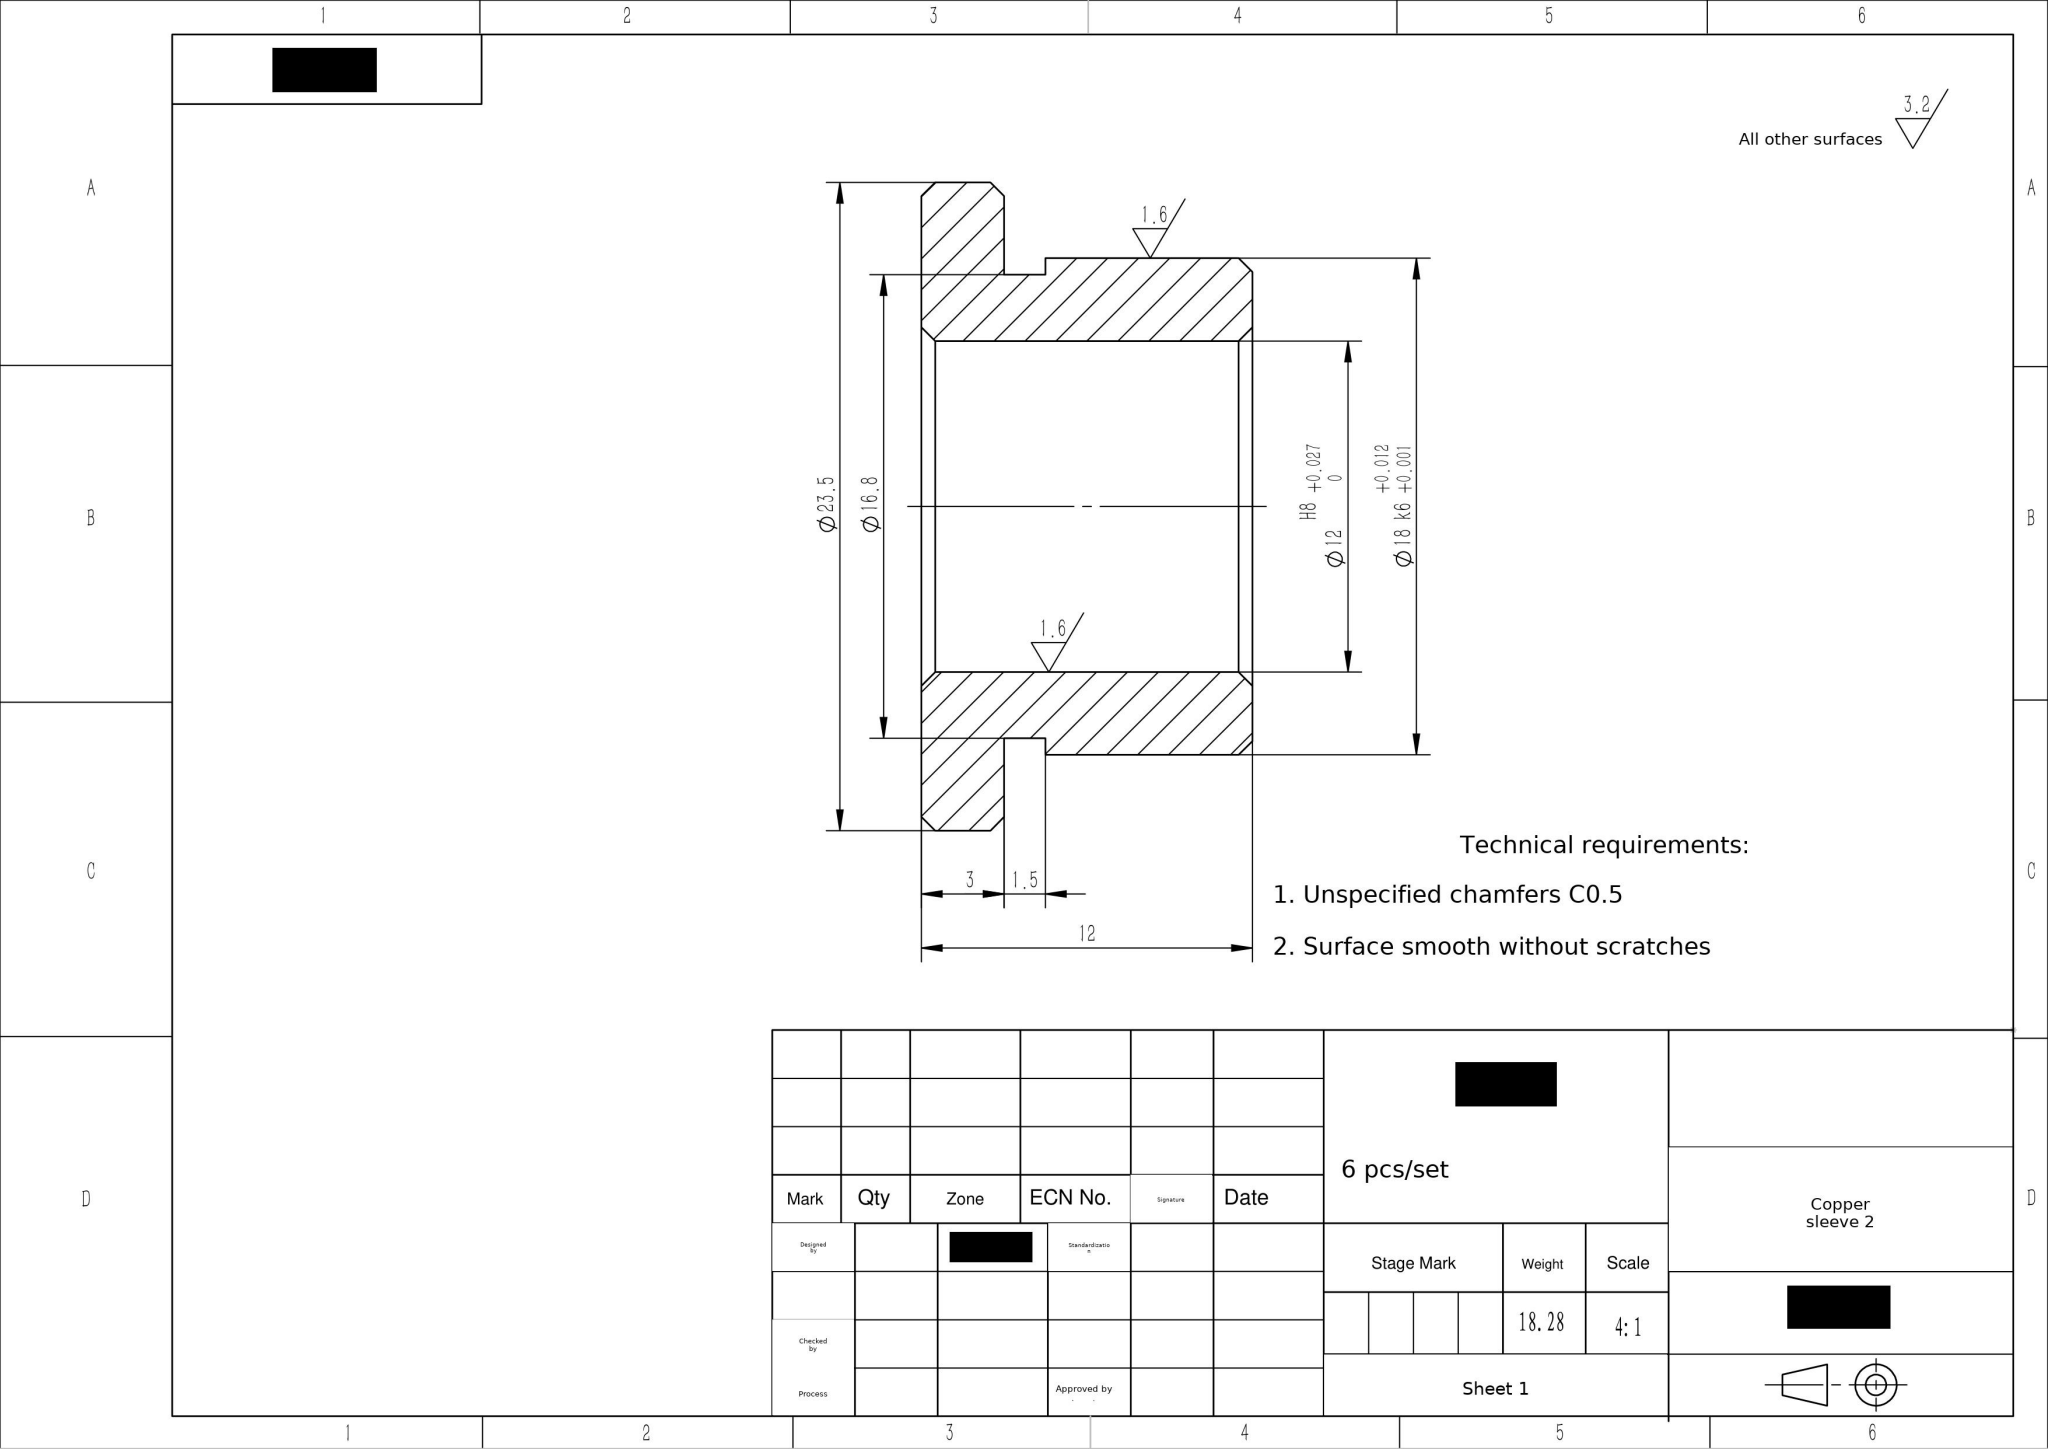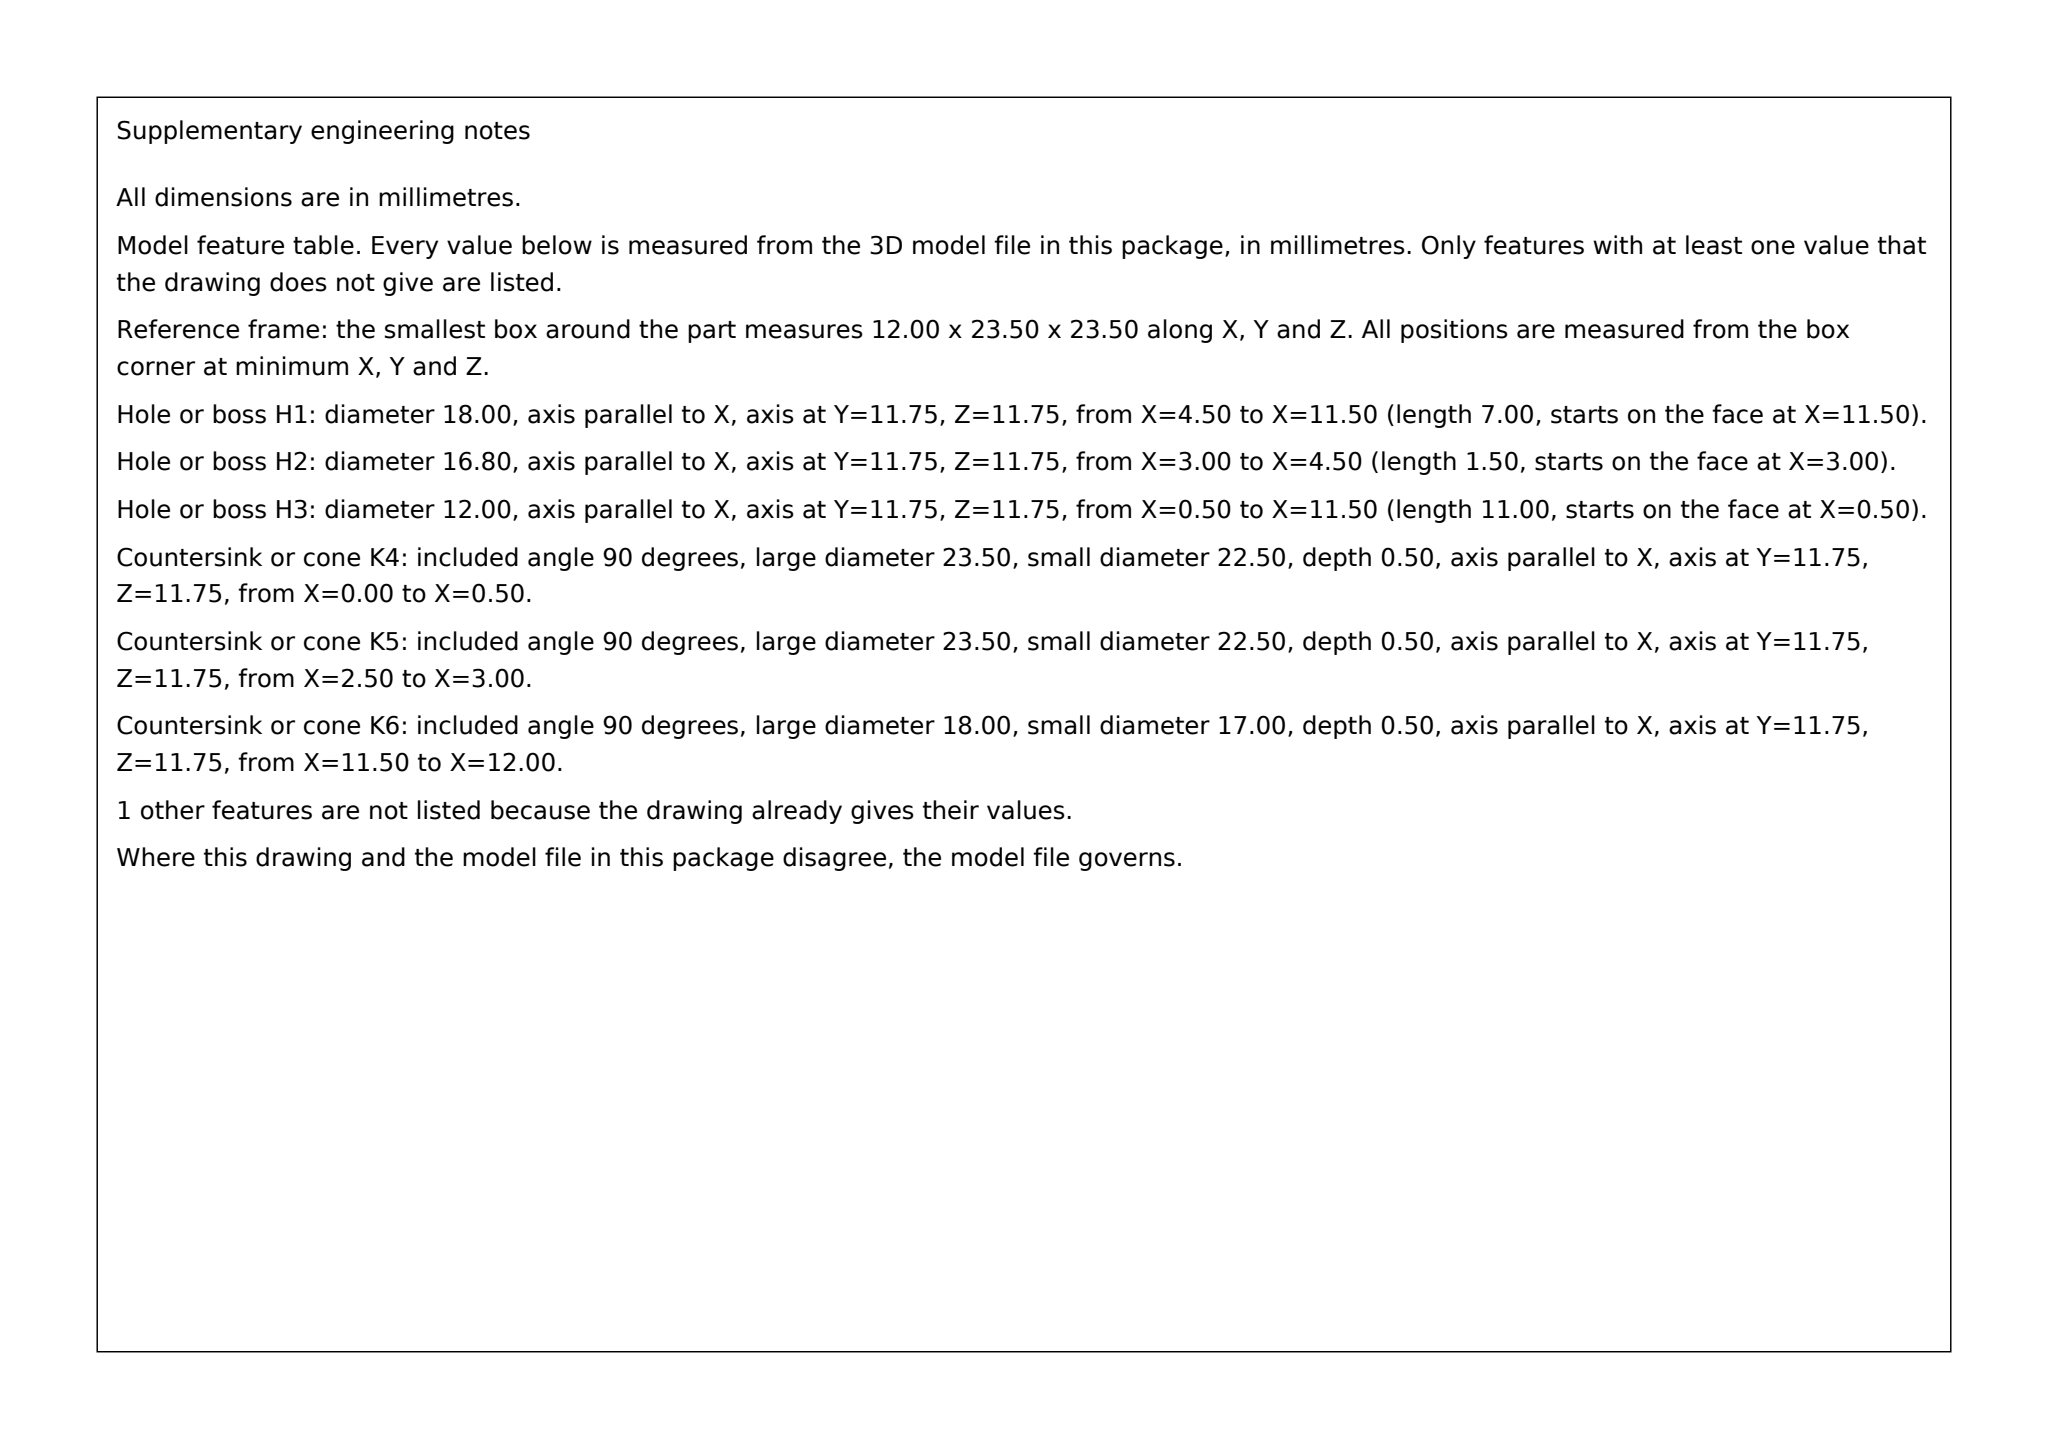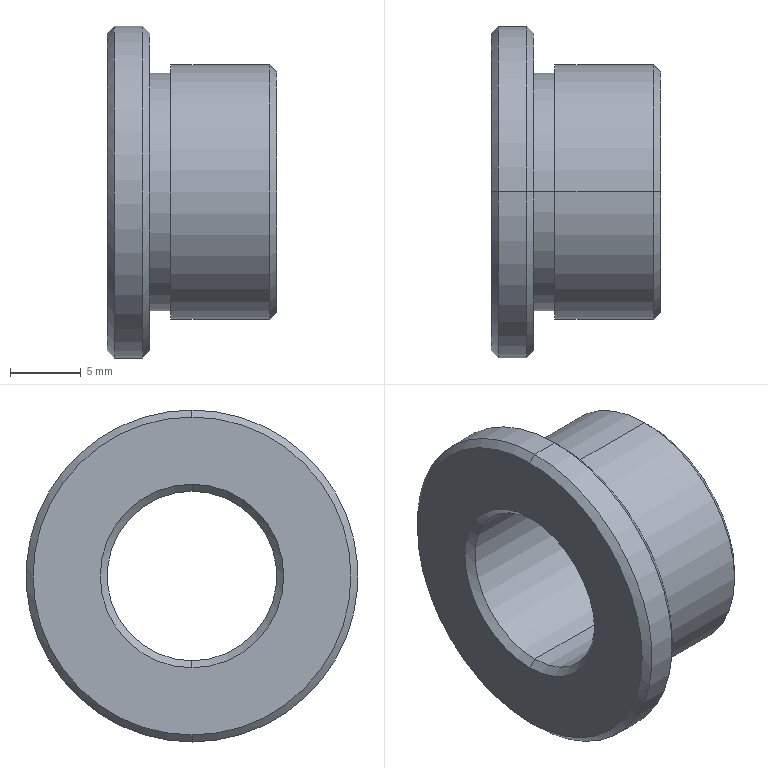Part | SolidWorks | mm | material Copper | 1 solid | 22 faces | box 12 x 23.5 x 23.5 mm | volume 2150 mm3 | cone 10 | cylinder 8 | plane 4 | commonest cylinder face diameters 16.8 x2 23.5 x2 18 x2 12 x2
build123d program:
from build123d import *

# Parameters (mm, degrees)
SKETCH1_W     = 12
SKETCH1_H     = 3
SKETCH2_W     = 3
SKETCH2_H     = 5.75
SKETCH3_W     = 1.5
SKETCH3_H     = 0.6
CHAMFER2_SIZE = 0.5


with BuildPart() as part:
    # Sketch1 → Revolve1 (revolve)
    with BuildSketch(Plane.XY, mode=Mode.PRIVATE) as revolve1_sk:
        with Locations((6, 7.5)):
            Rectangle(SKETCH1_W, SKETCH1_H)
    revolve(revolve1_sk.sketch.rotate(Axis((-11.601, 0, 0), (1, 0, 0)), 90), axis=Axis((-11.601, 0, 0), (1, 0, 0)))

    # Sketch2 → Revolve2 (revolve)
    with BuildSketch(Plane.XY, mode=Mode.PRIVATE) as revolve2_sk:
        with Locations((1.5, 8.875)):
            Rectangle(SKETCH2_W, SKETCH2_H)
    revolve(revolve2_sk.sketch.rotate(Axis((29.844, 0, 0), (-1, 0, 0)), 270), axis=Axis((29.844, 0, 0), (-1, 0, 0)))

    # Sketch3 → Cut-Revolve1 (revolve, cut)
    with BuildSketch(Plane.XY, mode=Mode.PRIVATE) as cut_revolve1_sk:
        with Locations((3.75, 8.7)):
            Rectangle(SKETCH3_W, SKETCH3_H)
    revolve(cut_revolve1_sk.sketch.rotate(Axis((16.33, 0, 0), (-1, 0, 0)), 90), axis=Axis((16.33, 0, 0), (-1, 0, 0)), mode=Mode.SUBTRACT)

    # Chamfer2
    chamfer2_edges = [part.edges().sort_by_distance(p)[0] for p in [
        (3, 0, -11.75),
        (0, 0, -11.75),
        (12, 0, -9),
        (12, 0, -6),
        (0, 0, -6),
    ]]
    chamfer(chamfer2_edges, length=CHAMFER2_SIZE)


solid = part.part
STEP:
#1=CARTESIAN_POINT('',(11.5,0.,6.));
#2=VERTEX_POINT('',#1);
#3=CARTESIAN_POINT('',(11.5,0.,-6.));
#4=VERTEX_POINT('',#3);
#5=CARTESIAN_POINT('',(11.5,0.,0.));
#6=DIRECTION('',(1.,0.,0.));
#7=DIRECTION('',(0.,0.,1.));
#8=AXIS2_PLACEMENT_3D('',#5,#6,#7);
#9=CIRCLE('',#8,6.);
#10=EDGE_CURVE('',#2,#4,#9,.T.);
#11=ORIENTED_EDGE('',*,*,#10,.F.);
#12=CARTESIAN_POINT('',(12.,0.,6.5));
#13=VERTEX_POINT('',#12);
#14=CARTESIAN_POINT('',(12.,0.,6.5));
#15=DIRECTION('',(0.7071,0.,0.7071));
#16=VECTOR('',#15,1000.);
#17=LINE('',#14,#16);
#18=EDGE_CURVE('',#2,#13,#17,.T.);
#19=ORIENTED_EDGE('',*,*,#18,.T.);
#20=CARTESIAN_POINT('',(12.,0.,-6.5));
#21=VERTEX_POINT('',#20);
#22=CARTESIAN_POINT('',(12.,0.,0.));
#23=DIRECTION('',(-1.,0.,0.));
#24=DIRECTION('',(0.,0.,1.));
#25=AXIS2_PLACEMENT_3D('',#22,#23,#24);
#26=CIRCLE('',#25,6.5);
#27=EDGE_CURVE('',#21,#13,#26,.T.);
#28=ORIENTED_EDGE('',*,*,#27,.F.);
#29=CARTESIAN_POINT('',(12.,0.,-6.5));
#30=DIRECTION('',(0.7071,0.,-0.7071));
#31=VECTOR('',#30,1000.);
#32=LINE('',#29,#31);
#33=EDGE_CURVE('',#4,#21,#32,.T.);
#34=ORIENTED_EDGE('',*,*,#33,.F.);
#35=EDGE_LOOP('',(#11,#19,#28,#34));
#36=FACE_OUTER_BOUND('',#35,.T.);
#37=CARTESIAN_POINT('',(12.,0.,0.));
#38=DIRECTION('',(1.,0.,0.));
#39=DIRECTION('',(0.,0.,-1.));
#40=AXIS2_PLACEMENT_3D('',#37,#38,#39);
#41=CONICAL_SURFACE('',#40,6.5,0.7854);
#42=ADVANCED_FACE('',(#36),#41,.F.);
#43=CARTESIAN_POINT('',(0.5,0.,-6.));
#44=VERTEX_POINT('',#43);
#45=CARTESIAN_POINT('',(0.5,0.,6.));
#46=VERTEX_POINT('',#45);
#47=CARTESIAN_POINT('',(0.5,0.,0.));
#48=DIRECTION('',(-1.,0.,0.));
#49=DIRECTION('',(0.,0.,-1.));
#50=AXIS2_PLACEMENT_3D('',#47,#48,#49);
#51=CIRCLE('',#50,6.);
#52=EDGE_CURVE('',#44,#46,#51,.T.);
#53=ORIENTED_EDGE('',*,*,#52,.F.);
#54=CARTESIAN_POINT('',(0.,0.,-6.5));
#55=VERTEX_POINT('',#54);
#56=CARTESIAN_POINT('',(0.5,0.,-6.));
#57=DIRECTION('',(-0.7071,0.,-0.7071));
#58=VECTOR('',#57,1000.);
#59=LINE('',#56,#58);
#60=EDGE_CURVE('',#44,#55,#59,.T.);
#61=ORIENTED_EDGE('',*,*,#60,.T.);
#62=CARTESIAN_POINT('',(0.,0.,6.5));
#63=VERTEX_POINT('',#62);
#64=CARTESIAN_POINT('',(0.,0.,0.));
#65=DIRECTION('',(1.,0.,0.));
#66=DIRECTION('',(0.,0.,-1.));
#67=AXIS2_PLACEMENT_3D('',#64,#65,#66);
#68=CIRCLE('',#67,6.5);
#69=EDGE_CURVE('',#63,#55,#68,.T.);
#70=ORIENTED_EDGE('',*,*,#69,.F.);
#71=CARTESIAN_POINT('',(0.5,0.,6.));
#72=DIRECTION('',(-0.7071,0.,0.7071));
#73=VECTOR('',#72,1000.);
#74=LINE('',#71,#73);
#75=EDGE_CURVE('',#46,#63,#74,.T.);
#76=ORIENTED_EDGE('',*,*,#75,.F.);
#77=EDGE_LOOP('',(#53,#61,#70,#76));
#78=FACE_OUTER_BOUND('',#77,.T.);
#79=CARTESIAN_POINT('',(0.5,0.,0.));
#80=DIRECTION('',(-1.,0.,0.));
#81=DIRECTION('',(0.,0.,1.));
#82=AXIS2_PLACEMENT_3D('',#79,#80,#81);
#83=CONICAL_SURFACE('',#82,6.,0.7854);
#84=ADVANCED_FACE('',(#78),#83,.F.);
#85=CARTESIAN_POINT('',(0.,0.,11.25));
#86=VERTEX_POINT('',#85);
#87=CARTESIAN_POINT('',(0.,0.,-11.25));
#88=VERTEX_POINT('',#87);
#89=CARTESIAN_POINT('',(0.,0.,0.));
#90=DIRECTION('',(-1.,0.,0.));
#91=DIRECTION('',(0.,0.,-1.));
#92=AXIS2_PLACEMENT_3D('',#89,#90,#91);
#93=CIRCLE('',#92,11.25);
#94=EDGE_CURVE('',#86,#88,#93,.T.);
#95=ORIENTED_EDGE('',*,*,#94,.F.);
#96=CARTESIAN_POINT('',(0.5,0.,11.75));
#97=VERTEX_POINT('',#96);
#98=CARTESIAN_POINT('',(0.5,0.,11.75));
#99=DIRECTION('',(0.7071,0.,0.7071));
#100=VECTOR('',#99,1000.);
#101=LINE('',#98,#100);
#102=EDGE_CURVE('',#86,#97,#101,.T.);
#103=ORIENTED_EDGE('',*,*,#102,.T.);
#104=CARTESIAN_POINT('',(0.5,0.,-11.75));
#105=VERTEX_POINT('',#104);
#106=CARTESIAN_POINT('',(0.5,0.,0.));
#107=DIRECTION('',(1.,0.,0.));
#108=DIRECTION('',(0.,0.,-1.));
#109=AXIS2_PLACEMENT_3D('',#106,#107,#108);
#110=CIRCLE('',#109,11.75);
#111=EDGE_CURVE('',#105,#97,#110,.T.);
#112=ORIENTED_EDGE('',*,*,#111,.F.);
#113=CARTESIAN_POINT('',(0.5,0.,-11.75));
#114=DIRECTION('',(0.7071,0.,-0.7071));
#115=VECTOR('',#114,1000.);
#116=LINE('',#113,#115);
#117=EDGE_CURVE('',#88,#105,#116,.T.);
#118=ORIENTED_EDGE('',*,*,#117,.F.);
#119=EDGE_LOOP('',(#95,#103,#112,#118));
#120=FACE_OUTER_BOUND('',#119,.T.);
#121=CARTESIAN_POINT('',(0.5,0.,0.));
#122=DIRECTION('',(1.,0.,0.));
#123=DIRECTION('',(0.,0.,-1.));
#124=AXIS2_PLACEMENT_3D('',#121,#122,#123);
#125=CONICAL_SURFACE('',#124,11.75,0.7854);
#126=ADVANCED_FACE('',(#120),#125,.T.);
#127=CARTESIAN_POINT('',(3.,0.,-11.25));
#128=VERTEX_POINT('',#127);
#129=CARTESIAN_POINT('',(3.,0.,11.25));
#130=VERTEX_POINT('',#129);
#131=CARTESIAN_POINT('',(3.,0.,0.));
#132=DIRECTION('',(1.,0.,0.));
#133=DIRECTION('',(0.,0.,-1.));
#134=AXIS2_PLACEMENT_3D('',#131,#132,#133);
#135=CIRCLE('',#134,11.25);
#136=EDGE_CURVE('',#128,#130,#135,.T.);
#137=ORIENTED_EDGE('',*,*,#136,.F.);
#138=CARTESIAN_POINT('',(2.5,0.,-11.75));
#139=VERTEX_POINT('',#138);
#140=CARTESIAN_POINT('',(3.,0.,-11.25));
#141=DIRECTION('',(-0.7071,0.,-0.7071));
#142=VECTOR('',#141,1000.);
#143=LINE('',#140,#142);
#144=EDGE_CURVE('',#128,#139,#143,.T.);
#145=ORIENTED_EDGE('',*,*,#144,.T.);
#146=CARTESIAN_POINT('',(2.5,0.,11.75));
#147=VERTEX_POINT('',#146);
#148=CARTESIAN_POINT('',(2.5,0.,0.));
#149=DIRECTION('',(-1.,0.,0.));
#150=DIRECTION('',(0.,0.,-1.));
#151=AXIS2_PLACEMENT_3D('',#148,#149,#150);
#152=CIRCLE('',#151,11.75);
#153=EDGE_CURVE('',#147,#139,#152,.T.);
#154=ORIENTED_EDGE('',*,*,#153,.F.);
#155=CARTESIAN_POINT('',(3.,0.,11.25));
#156=DIRECTION('',(-0.7071,0.,0.7071));
#157=VECTOR('',#156,1000.);
#158=LINE('',#155,#157);
#159=EDGE_CURVE('',#130,#147,#158,.T.);
#160=ORIENTED_EDGE('',*,*,#159,.F.);
#161=EDGE_LOOP('',(#137,#145,#154,#160));
#162=FACE_OUTER_BOUND('',#161,.T.);
#163=CARTESIAN_POINT('',(3.,0.,0.));
#164=DIRECTION('',(-1.,0.,0.));
#165=DIRECTION('',(0.,0.,1.));
#166=AXIS2_PLACEMENT_3D('',#163,#164,#165);
#167=CONICAL_SURFACE('',#166,11.25,0.7854);
#168=ADVANCED_FACE('',(#162),#167,.T.);
#169=CARTESIAN_POINT('',(12.,0.,-8.5));
#170=VERTEX_POINT('',#169);
#171=CARTESIAN_POINT('',(12.,0.,8.5));
#172=VERTEX_POINT('',#171);
#173=CARTESIAN_POINT('',(12.,0.,0.));
#174=DIRECTION('',(1.,0.,0.));
#175=DIRECTION('',(0.,0.,1.));
#176=AXIS2_PLACEMENT_3D('',#173,#174,#175);
#177=CIRCLE('',#176,8.5);
#178=EDGE_CURVE('',#170,#172,#177,.T.);
#179=ORIENTED_EDGE('',*,*,#178,.F.);
#180=CARTESIAN_POINT('',(11.5,0.,-9.));
#181=VERTEX_POINT('',#180);
#182=CARTESIAN_POINT('',(11.5,0.,-9.));
#183=DIRECTION('',(-0.7071,0.,-0.7071));
#184=VECTOR('',#183,1000.);
#185=LINE('',#182,#184);
#186=EDGE_CURVE('',#170,#181,#185,.T.);
#187=ORIENTED_EDGE('',*,*,#186,.T.);
#188=CARTESIAN_POINT('',(11.5,0.,9.));
#189=VERTEX_POINT('',#188);
#190=CARTESIAN_POINT('',(11.5,0.,0.));
#191=DIRECTION('',(-1.,0.,0.));
#192=DIRECTION('',(0.,0.,1.));
#193=AXIS2_PLACEMENT_3D('',#190,#191,#192);
#194=CIRCLE('',#193,9.);
#195=EDGE_CURVE('',#189,#181,#194,.T.);
#196=ORIENTED_EDGE('',*,*,#195,.F.);
#197=CARTESIAN_POINT('',(11.5,0.,9.));
#198=DIRECTION('',(-0.7071,0.,0.7071));
#199=VECTOR('',#198,1000.);
#200=LINE('',#197,#199);
#201=EDGE_CURVE('',#172,#189,#200,.T.);
#202=ORIENTED_EDGE('',*,*,#201,.F.);
#203=EDGE_LOOP('',(#179,#187,#196,#202));
#204=FACE_OUTER_BOUND('',#203,.T.);
#205=CARTESIAN_POINT('',(11.5,0.,0.));
#206=DIRECTION('',(-1.,0.,0.));
#207=DIRECTION('',(0.,0.,1.));
#208=AXIS2_PLACEMENT_3D('',#205,#206,#207);
#209=CONICAL_SURFACE('',#208,9.,0.7854);
#210=ADVANCED_FACE('',(#204),#209,.T.);
#211=CARTESIAN_POINT('',(3.,0.,-8.4));
#212=VERTEX_POINT('',#211);
#213=CARTESIAN_POINT('',(3.,0.,8.4));
#214=VERTEX_POINT('',#213);
#215=CARTESIAN_POINT('',(3.,0.,0.));
#216=DIRECTION('',(1.,0.,0.));
#217=DIRECTION('',(0.,0.,-1.));
#218=AXIS2_PLACEMENT_3D('',#215,#216,#217);
#219=CIRCLE('',#218,8.4);
#220=EDGE_CURVE('',#212,#214,#219,.T.);
#221=ORIENTED_EDGE('',*,*,#220,.T.);
#222=CARTESIAN_POINT('',(4.5,0.,8.4));
#223=VERTEX_POINT('',#222);
#224=CARTESIAN_POINT('',(16.33,0.,8.4));
#225=DIRECTION('',(1.,0.,0.));
#226=VECTOR('',#225,1000.);
#227=LINE('',#224,#226);
#228=EDGE_CURVE('',#214,#223,#227,.T.);
#229=ORIENTED_EDGE('',*,*,#228,.T.);
#230=CARTESIAN_POINT('',(4.5,0.,-8.4));
#231=VERTEX_POINT('',#230);
#232=CARTESIAN_POINT('',(4.5,0.,0.));
#233=DIRECTION('',(1.,0.,0.));
#234=DIRECTION('',(0.,0.,-1.));
#235=AXIS2_PLACEMENT_3D('',#232,#233,#234);
#236=CIRCLE('',#235,8.4);
#237=EDGE_CURVE('',#231,#223,#236,.T.);
#238=ORIENTED_EDGE('',*,*,#237,.F.);
#239=CARTESIAN_POINT('',(16.33,0.,-8.4));
#240=DIRECTION('',(1.,0.,0.));
#241=VECTOR('',#240,1000.);
#242=LINE('',#239,#241);
#243=EDGE_CURVE('',#212,#231,#242,.T.);
#244=ORIENTED_EDGE('',*,*,#243,.F.);
#245=EDGE_LOOP('',(#221,#229,#238,#244));
#246=FACE_OUTER_BOUND('',#245,.T.);
#247=CARTESIAN_POINT('',(16.33,0.,0.));
#248=DIRECTION('',(1.,0.,0.));
#249=DIRECTION('',(0.,0.,-1.));
#250=AXIS2_PLACEMENT_3D('',#247,#248,#249);
#251=CYLINDRICAL_SURFACE('',#250,8.4);
#252=ADVANCED_FACE('',(#246),#251,.T.);
#253=ORIENTED_EDGE('',*,*,#111,.T.);
#254=CARTESIAN_POINT('',(29.844,0.,11.75));
#255=DIRECTION('',(1.,0.,0.));
#256=VECTOR('',#255,1000.);
#257=LINE('',#254,#256);
#258=EDGE_CURVE('',#97,#147,#257,.T.);
#259=ORIENTED_EDGE('',*,*,#258,.T.);
#260=ORIENTED_EDGE('',*,*,#153,.T.);
#261=CARTESIAN_POINT('',(29.844,0.,-11.75));
#262=DIRECTION('',(1.,0.,0.));
#263=VECTOR('',#262,1000.);
#264=LINE('',#261,#263);
#265=EDGE_CURVE('',#105,#139,#264,.T.);
#266=ORIENTED_EDGE('',*,*,#265,.F.);
#267=EDGE_LOOP('',(#253,#259,#260,#266));
#268=FACE_OUTER_BOUND('',#267,.T.);
#269=CARTESIAN_POINT('',(29.844,0.,0.));
#270=DIRECTION('',(1.,0.,0.));
#271=DIRECTION('',(0.,0.,-1.));
#272=AXIS2_PLACEMENT_3D('',#269,#270,#271);
#273=CYLINDRICAL_SURFACE('',#272,11.75);
#274=ADVANCED_FACE('',(#268),#273,.T.);
#275=ORIENTED_EDGE('',*,*,#195,.T.);
#276=CARTESIAN_POINT('',(4.5,0.,-9.));
#277=VERTEX_POINT('',#276);
#278=CARTESIAN_POINT('',(-11.601,0.,-9.));
#279=DIRECTION('',(-1.,0.,0.));
#280=VECTOR('',#279,1000.);
#281=LINE('',#278,#280);
#282=EDGE_CURVE('',#181,#277,#281,.T.);
#283=ORIENTED_EDGE('',*,*,#282,.T.);
#284=CARTESIAN_POINT('',(4.5,0.,9.));
#285=VERTEX_POINT('',#284);
#286=CARTESIAN_POINT('',(4.5,0.,0.));
#287=DIRECTION('',(1.,0.,0.));
#288=DIRECTION('',(0.,0.,-1.));
#289=AXIS2_PLACEMENT_3D('',#286,#287,#288);
#290=CIRCLE('',#289,9.);
#291=EDGE_CURVE('',#277,#285,#290,.T.);
#292=ORIENTED_EDGE('',*,*,#291,.T.);
#293=CARTESIAN_POINT('',(-11.601,0.,9.));
#294=DIRECTION('',(-1.,0.,0.));
#295=VECTOR('',#294,1000.);
#296=LINE('',#293,#295);
#297=EDGE_CURVE('',#189,#285,#296,.T.);
#298=ORIENTED_EDGE('',*,*,#297,.F.);
#299=EDGE_LOOP('',(#275,#283,#292,#298));
#300=FACE_OUTER_BOUND('',#299,.T.);
#301=CARTESIAN_POINT('',(-11.601,0.,0.));
#302=DIRECTION('',(-1.,0.,0.));
#303=DIRECTION('',(0.,0.,1.));
#304=AXIS2_PLACEMENT_3D('',#301,#302,#303);
#305=CYLINDRICAL_SURFACE('',#304,9.);
#306=ADVANCED_FACE('',(#300),#305,.T.);
#307=ORIENTED_EDGE('',*,*,#10,.T.);
#308=CARTESIAN_POINT('',(-11.601,0.,-6.));
#309=DIRECTION('',(-1.,0.,0.));
#310=VECTOR('',#309,1000.);
#311=LINE('',#308,#310);
#312=EDGE_CURVE('',#4,#44,#311,.T.);
#313=ORIENTED_EDGE('',*,*,#312,.T.);
#314=ORIENTED_EDGE('',*,*,#52,.T.);
#315=CARTESIAN_POINT('',(-11.601,0.,6.));
#316=DIRECTION('',(-1.,0.,0.));
#317=VECTOR('',#316,1000.);
#318=LINE('',#315,#317);
#319=EDGE_CURVE('',#2,#46,#318,.T.);
#320=ORIENTED_EDGE('',*,*,#319,.F.);
#321=EDGE_LOOP('',(#307,#313,#314,#320));
#322=FACE_OUTER_BOUND('',#321,.T.);
#323=CARTESIAN_POINT('',(-11.601,0.,0.));
#324=DIRECTION('',(-1.,0.,0.));
#325=DIRECTION('',(0.,0.,1.));
#326=AXIS2_PLACEMENT_3D('',#323,#324,#325);
#327=CYLINDRICAL_SURFACE('',#326,6.);
#328=ADVANCED_FACE('',(#322),#327,.F.);
#329=CARTESIAN_POINT('',(0.,0.,0.));
#330=DIRECTION('',(-1.,0.,0.));
#331=DIRECTION('',(0.,0.,-1.));
#332=AXIS2_PLACEMENT_3D('',#329,#330,#331);
#333=CIRCLE('',#332,11.25);
#334=EDGE_CURVE('',#88,#86,#333,.T.);
#335=ORIENTED_EDGE('',*,*,#334,.T.);
#336=ORIENTED_EDGE('',*,*,#94,.T.);
#337=EDGE_LOOP('',(#335,#336));
#338=FACE_OUTER_BOUND('',#337,.T.);
#339=ORIENTED_EDGE('',*,*,#69,.T.);
#340=CARTESIAN_POINT('',(0.,0.,0.));
#341=DIRECTION('',(1.,0.,0.));
#342=DIRECTION('',(0.,0.,-1.));
#343=AXIS2_PLACEMENT_3D('',#340,#341,#342);
#344=CIRCLE('',#343,6.5);
#345=EDGE_CURVE('',#55,#63,#344,.T.);
#346=ORIENTED_EDGE('',*,*,#345,.T.);
#347=EDGE_LOOP('',(#339,#346));
#348=FACE_BOUND('',#347,.T.);
#349=CARTESIAN_POINT('',(0.,9.,0.));
#350=DIRECTION('',(1.,0.,0.));
#351=DIRECTION('',(0.,0.,-1.));
#352=AXIS2_PLACEMENT_3D('',#349,#350,#351);
#353=PLANE('',#352);
#354=ADVANCED_FACE('',(#338,#348),#353,.F.);
#355=ORIENTED_EDGE('',*,*,#312,.F.);
#356=CARTESIAN_POINT('',(11.5,0.,0.));
#357=DIRECTION('',(1.,0.,0.));
#358=DIRECTION('',(0.,0.,1.));
#359=AXIS2_PLACEMENT_3D('',#356,#357,#358);
#360=CIRCLE('',#359,6.);
#361=EDGE_CURVE('',#4,#2,#360,.T.);
#362=ORIENTED_EDGE('',*,*,#361,.T.);
#363=ORIENTED_EDGE('',*,*,#319,.T.);
#364=CARTESIAN_POINT('',(0.5,0.,0.));
#365=DIRECTION('',(-1.,0.,0.));
#366=DIRECTION('',(0.,0.,-1.));
#367=AXIS2_PLACEMENT_3D('',#364,#365,#366);
#368=CIRCLE('',#367,6.);
#369=EDGE_CURVE('',#46,#44,#368,.T.);
#370=ORIENTED_EDGE('',*,*,#369,.T.);
#371=EDGE_LOOP('',(#355,#362,#363,#370));
#372=FACE_OUTER_BOUND('',#371,.T.);
#373=CARTESIAN_POINT('',(-11.601,0.,0.));
#374=DIRECTION('',(-1.,0.,0.));
#375=DIRECTION('',(0.,0.,1.));
#376=AXIS2_PLACEMENT_3D('',#373,#374,#375);
#377=CYLINDRICAL_SURFACE('',#376,6.);
#378=ADVANCED_FACE('',(#372),#377,.F.);
#379=CARTESIAN_POINT('',(12.,0.,0.));
#380=DIRECTION('',(1.,0.,0.));
#381=DIRECTION('',(0.,0.,1.));
#382=AXIS2_PLACEMENT_3D('',#379,#380,#381);
#383=CIRCLE('',#382,8.5);
#384=EDGE_CURVE('',#172,#170,#383,.T.);
#385=ORIENTED_EDGE('',*,*,#384,.T.);
#386=ORIENTED_EDGE('',*,*,#178,.T.);
#387=EDGE_LOOP('',(#385,#386));
#388=FACE_OUTER_BOUND('',#387,.T.);
#389=ORIENTED_EDGE('',*,*,#27,.T.);
#390=CARTESIAN_POINT('',(12.,0.,0.));
#391=DIRECTION('',(-1.,0.,0.));
#392=DIRECTION('',(0.,0.,1.));
#393=AXIS2_PLACEMENT_3D('',#390,#391,#392);
#394=CIRCLE('',#393,6.5);
#395=EDGE_CURVE('',#13,#21,#394,.T.);
#396=ORIENTED_EDGE('',*,*,#395,.T.);
#397=EDGE_LOOP('',(#389,#396));
#398=FACE_BOUND('',#397,.T.);
#399=CARTESIAN_POINT('',(12.,9.,0.));
#400=DIRECTION('',(-1.,0.,0.));
#401=DIRECTION('',(0.,0.,1.));
#402=AXIS2_PLACEMENT_3D('',#399,#400,#401);
#403=PLANE('',#402);
#404=ADVANCED_FACE('',(#388,#398),#403,.F.);
#405=ORIENTED_EDGE('',*,*,#282,.F.);
#406=CARTESIAN_POINT('',(11.5,0.,0.));
#407=DIRECTION('',(-1.,0.,0.));
#408=DIRECTION('',(0.,0.,1.));
#409=AXIS2_PLACEMENT_3D('',#406,#407,#408);
#410=CIRCLE('',#409,9.);
#411=EDGE_CURVE('',#181,#189,#410,.T.);
#412=ORIENTED_EDGE('',*,*,#411,.T.);
#413=ORIENTED_EDGE('',*,*,#297,.T.);
#414=CARTESIAN_POINT('',(4.5,0.,0.));
#415=DIRECTION('',(1.,0.,0.));
#416=DIRECTION('',(0.,0.,-1.));
#417=AXIS2_PLACEMENT_3D('',#414,#415,#416);
#418=CIRCLE('',#417,9.);
#419=EDGE_CURVE('',#285,#277,#418,.T.);
#420=ORIENTED_EDGE('',*,*,#419,.T.);
#421=EDGE_LOOP('',(#405,#412,#413,#420));
#422=FACE_OUTER_BOUND('',#421,.T.);
#423=CARTESIAN_POINT('',(-11.601,0.,0.));
#424=DIRECTION('',(-1.,0.,0.));
#425=DIRECTION('',(0.,0.,1.));
#426=AXIS2_PLACEMENT_3D('',#423,#424,#425);
#427=CYLINDRICAL_SURFACE('',#426,9.);
#428=ADVANCED_FACE('',(#422),#427,.T.);
#429=CARTESIAN_POINT('',(3.,0.,0.));
#430=DIRECTION('',(1.,0.,0.));
#431=DIRECTION('',(0.,0.,-1.));
#432=AXIS2_PLACEMENT_3D('',#429,#430,#431);
#433=CIRCLE('',#432,11.25);
#434=EDGE_CURVE('',#130,#128,#433,.T.);
#435=ORIENTED_EDGE('',*,*,#434,.T.);
#436=ORIENTED_EDGE('',*,*,#136,.T.);
#437=EDGE_LOOP('',(#435,#436));
#438=FACE_OUTER_BOUND('',#437,.T.);
#439=ORIENTED_EDGE('',*,*,#220,.F.);
#440=CARTESIAN_POINT('',(3.,0.,0.));
#441=DIRECTION('',(1.,0.,0.));
#442=DIRECTION('',(0.,0.,-1.));
#443=AXIS2_PLACEMENT_3D('',#440,#441,#442);
#444=CIRCLE('',#443,8.4);
#445=EDGE_CURVE('',#214,#212,#444,.T.);
#446=ORIENTED_EDGE('',*,*,#445,.F.);
#447=EDGE_LOOP('',(#439,#446));
#448=FACE_BOUND('',#447,.T.);
#449=CARTESIAN_POINT('',(3.,6.,0.));
#450=DIRECTION('',(1.,0.,0.));
#451=DIRECTION('',(0.,0.,-1.));
#452=AXIS2_PLACEMENT_3D('',#449,#450,#451);
#453=PLANE('',#452);
#454=ADVANCED_FACE('',(#438,#448),#453,.T.);
#455=ORIENTED_EDGE('',*,*,#258,.F.);
#456=CARTESIAN_POINT('',(0.5,0.,0.));
#457=DIRECTION('',(1.,0.,0.));
#458=DIRECTION('',(0.,0.,-1.));
#459=AXIS2_PLACEMENT_3D('',#456,#457,#458);
#460=CIRCLE('',#459,11.75);
#461=EDGE_CURVE('',#97,#105,#460,.T.);
#462=ORIENTED_EDGE('',*,*,#461,.T.);
#463=ORIENTED_EDGE('',*,*,#265,.T.);
#464=CARTESIAN_POINT('',(2.5,0.,0.));
#465=DIRECTION('',(-1.,0.,0.));
#466=DIRECTION('',(0.,0.,-1.));
#467=AXIS2_PLACEMENT_3D('',#464,#465,#466);
#468=CIRCLE('',#467,11.75);
#469=EDGE_CURVE('',#139,#147,#468,.T.);
#470=ORIENTED_EDGE('',*,*,#469,.T.);
#471=EDGE_LOOP('',(#455,#462,#463,#470));
#472=FACE_OUTER_BOUND('',#471,.T.);
#473=CARTESIAN_POINT('',(29.844,0.,0.));
#474=DIRECTION('',(1.,0.,0.));
#475=DIRECTION('',(0.,0.,-1.));
#476=AXIS2_PLACEMENT_3D('',#473,#474,#475);
#477=CYLINDRICAL_SURFACE('',#476,11.75);
#478=ADVANCED_FACE('',(#472),#477,.T.);
#479=ORIENTED_EDGE('',*,*,#228,.F.);
#480=ORIENTED_EDGE('',*,*,#445,.T.);
#481=ORIENTED_EDGE('',*,*,#243,.T.);
#482=CARTESIAN_POINT('',(4.5,0.,0.));
#483=DIRECTION('',(1.,0.,0.));
#484=DIRECTION('',(0.,0.,-1.));
#485=AXIS2_PLACEMENT_3D('',#482,#483,#484);
#486=CIRCLE('',#485,8.4);
#487=EDGE_CURVE('',#223,#231,#486,.T.);
#488=ORIENTED_EDGE('',*,*,#487,.F.);
#489=EDGE_LOOP('',(#479,#480,#481,#488));
#490=FACE_OUTER_BOUND('',#489,.T.);
#491=CARTESIAN_POINT('',(16.33,0.,0.));
#492=DIRECTION('',(1.,0.,0.));
#493=DIRECTION('',(0.,0.,-1.));
#494=AXIS2_PLACEMENT_3D('',#491,#492,#493);
#495=CYLINDRICAL_SURFACE('',#494,8.4);
#496=ADVANCED_FACE('',(#490),#495,.T.);
#497=ORIENTED_EDGE('',*,*,#419,.F.);
#498=ORIENTED_EDGE('',*,*,#291,.F.);
#499=EDGE_LOOP('',(#497,#498));
#500=FACE_OUTER_BOUND('',#499,.T.);
#501=ORIENTED_EDGE('',*,*,#237,.T.);
#502=ORIENTED_EDGE('',*,*,#487,.T.);
#503=EDGE_LOOP('',(#501,#502));
#504=FACE_BOUND('',#503,.T.);
#505=CARTESIAN_POINT('',(4.5,9.,0.));
#506=DIRECTION('',(1.,0.,0.));
#507=DIRECTION('',(0.,0.,-1.));
#508=AXIS2_PLACEMENT_3D('',#505,#506,#507);
#509=PLANE('',#508);
#510=ADVANCED_FACE('',(#500,#504),#509,.F.);
#511=ORIENTED_EDGE('',*,*,#186,.F.);
#512=ORIENTED_EDGE('',*,*,#384,.F.);
#513=ORIENTED_EDGE('',*,*,#201,.T.);
#514=ORIENTED_EDGE('',*,*,#411,.F.);
#515=EDGE_LOOP('',(#511,#512,#513,#514));
#516=FACE_OUTER_BOUND('',#515,.T.);
#517=CARTESIAN_POINT('',(11.5,0.,0.));
#518=DIRECTION('',(-1.,0.,0.));
#519=DIRECTION('',(0.,0.,1.));
#520=AXIS2_PLACEMENT_3D('',#517,#518,#519);
#521=CONICAL_SURFACE('',#520,9.,0.7854);
#522=ADVANCED_FACE('',(#516),#521,.T.);
#523=ORIENTED_EDGE('',*,*,#144,.F.);
#524=ORIENTED_EDGE('',*,*,#434,.F.);
#525=ORIENTED_EDGE('',*,*,#159,.T.);
#526=ORIENTED_EDGE('',*,*,#469,.F.);
#527=EDGE_LOOP('',(#523,#524,#525,#526));
#528=FACE_OUTER_BOUND('',#527,.T.);
#529=CARTESIAN_POINT('',(3.,0.,0.));
#530=DIRECTION('',(-1.,0.,0.));
#531=DIRECTION('',(0.,0.,1.));
#532=AXIS2_PLACEMENT_3D('',#529,#530,#531);
#533=CONICAL_SURFACE('',#532,11.25,0.7854);
#534=ADVANCED_FACE('',(#528),#533,.T.);
#535=ORIENTED_EDGE('',*,*,#102,.F.);
#536=ORIENTED_EDGE('',*,*,#334,.F.);
#537=ORIENTED_EDGE('',*,*,#117,.T.);
#538=ORIENTED_EDGE('',*,*,#461,.F.);
#539=EDGE_LOOP('',(#535,#536,#537,#538));
#540=FACE_OUTER_BOUND('',#539,.T.);
#541=CARTESIAN_POINT('',(0.5,0.,0.));
#542=DIRECTION('',(1.,0.,0.));
#543=DIRECTION('',(0.,0.,-1.));
#544=AXIS2_PLACEMENT_3D('',#541,#542,#543);
#545=CONICAL_SURFACE('',#544,11.75,0.7854);
#546=ADVANCED_FACE('',(#540),#545,.T.);
#547=ORIENTED_EDGE('',*,*,#60,.F.);
#548=ORIENTED_EDGE('',*,*,#369,.F.);
#549=ORIENTED_EDGE('',*,*,#75,.T.);
#550=ORIENTED_EDGE('',*,*,#345,.F.);
#551=EDGE_LOOP('',(#547,#548,#549,#550));
#552=FACE_OUTER_BOUND('',#551,.T.);
#553=CARTESIAN_POINT('',(0.5,0.,0.));
#554=DIRECTION('',(-1.,0.,0.));
#555=DIRECTION('',(0.,0.,1.));
#556=AXIS2_PLACEMENT_3D('',#553,#554,#555);
#557=CONICAL_SURFACE('',#556,6.,0.7854);
#558=ADVANCED_FACE('',(#552),#557,.F.);
#559=ORIENTED_EDGE('',*,*,#18,.F.);
#560=ORIENTED_EDGE('',*,*,#361,.F.);
#561=ORIENTED_EDGE('',*,*,#33,.T.);
#562=ORIENTED_EDGE('',*,*,#395,.F.);
#563=EDGE_LOOP('',(#559,#560,#561,#562));
#564=FACE_OUTER_BOUND('',#563,.T.);
#565=CARTESIAN_POINT('',(12.,0.,0.));
#566=DIRECTION('',(1.,0.,0.));
#567=DIRECTION('',(0.,0.,-1.));
#568=AXIS2_PLACEMENT_3D('',#565,#566,#567);
#569=CONICAL_SURFACE('',#568,6.5,0.7854);
#570=ADVANCED_FACE('',(#564),#569,.F.);
#571=CLOSED_SHELL('',(#42,#84,#126,#168,#210,#252,#274,#306,#328,#354,#378,#404,#428,#454,#478,#496,#510,#522,#534,#546,#558,#570));
#572=MANIFOLD_SOLID_BREP('',#571);
#573=CARTESIAN_POINT('',(0.,0.,0.));
#574=DIRECTION('',(0.,0.,1.));
#575=DIRECTION('',(1.,0.,0.));
#576=AXIS2_PLACEMENT_3D('',#573,#574,#575);
#577=(LENGTH_UNIT()NAMED_UNIT(*)SI_UNIT(.MILLI.,.METRE.));
#578=UNCERTAINTY_MEASURE_WITH_UNIT(LENGTH_MEASURE(0.00001),#577,'','');
#579=(NAMED_UNIT(*)PLANE_ANGLE_UNIT()SI_UNIT($,.RADIAN.));
#580=(NAMED_UNIT(*)SI_UNIT($,.STERADIAN.)SOLID_ANGLE_UNIT());
#581=(GEOMETRIC_REPRESENTATION_CONTEXT(3)GLOBAL_UNCERTAINTY_ASSIGNED_CONTEXT((#578))GLOBAL_UNIT_ASSIGNED_CONTEXT((#577,#579,#580))REPRESENTATION_CONTEXT('',''));
#582=ADVANCED_BREP_SHAPE_REPRESENTATION('',(#572,#576),#581);